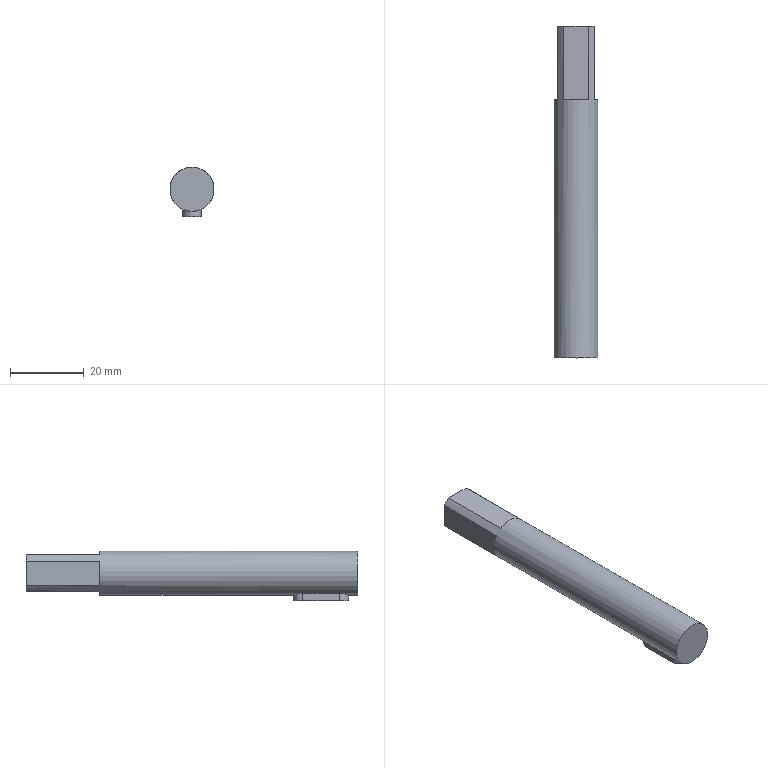Component | NX | SHAFT | 2 solids | 22 faces | volume 9935 mm3 | plane 17 | cylinder 5 | commonest cylinder face diameters 5 x4 12 x1